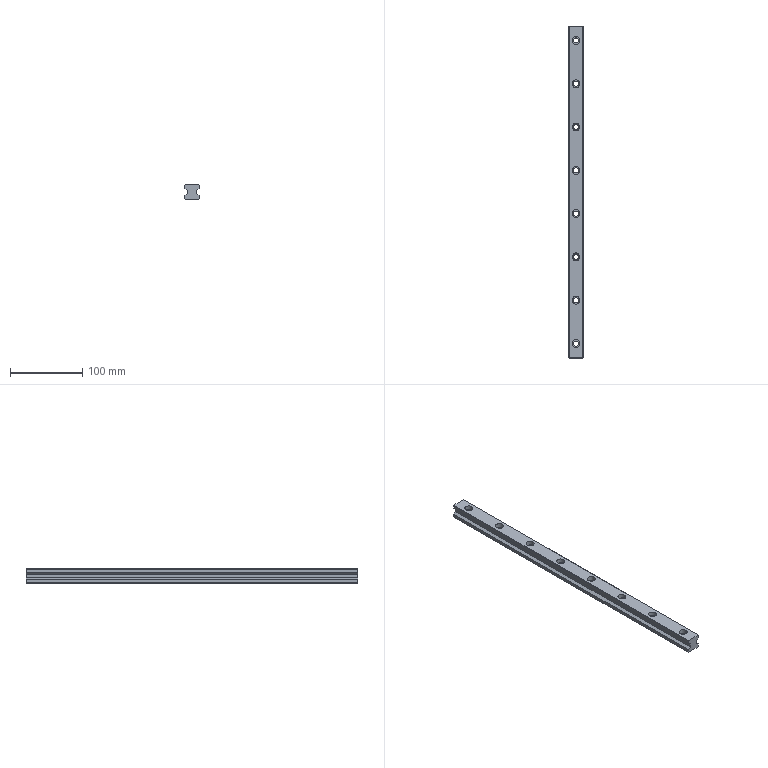Component | NX | LINEAR_CUTTER_RAIL_2 | 1 solid | 42 faces | volume 146597 mm3 | plane 26 | cylinder 16 | commonest cylinder face diameters 7 x8 11 x8